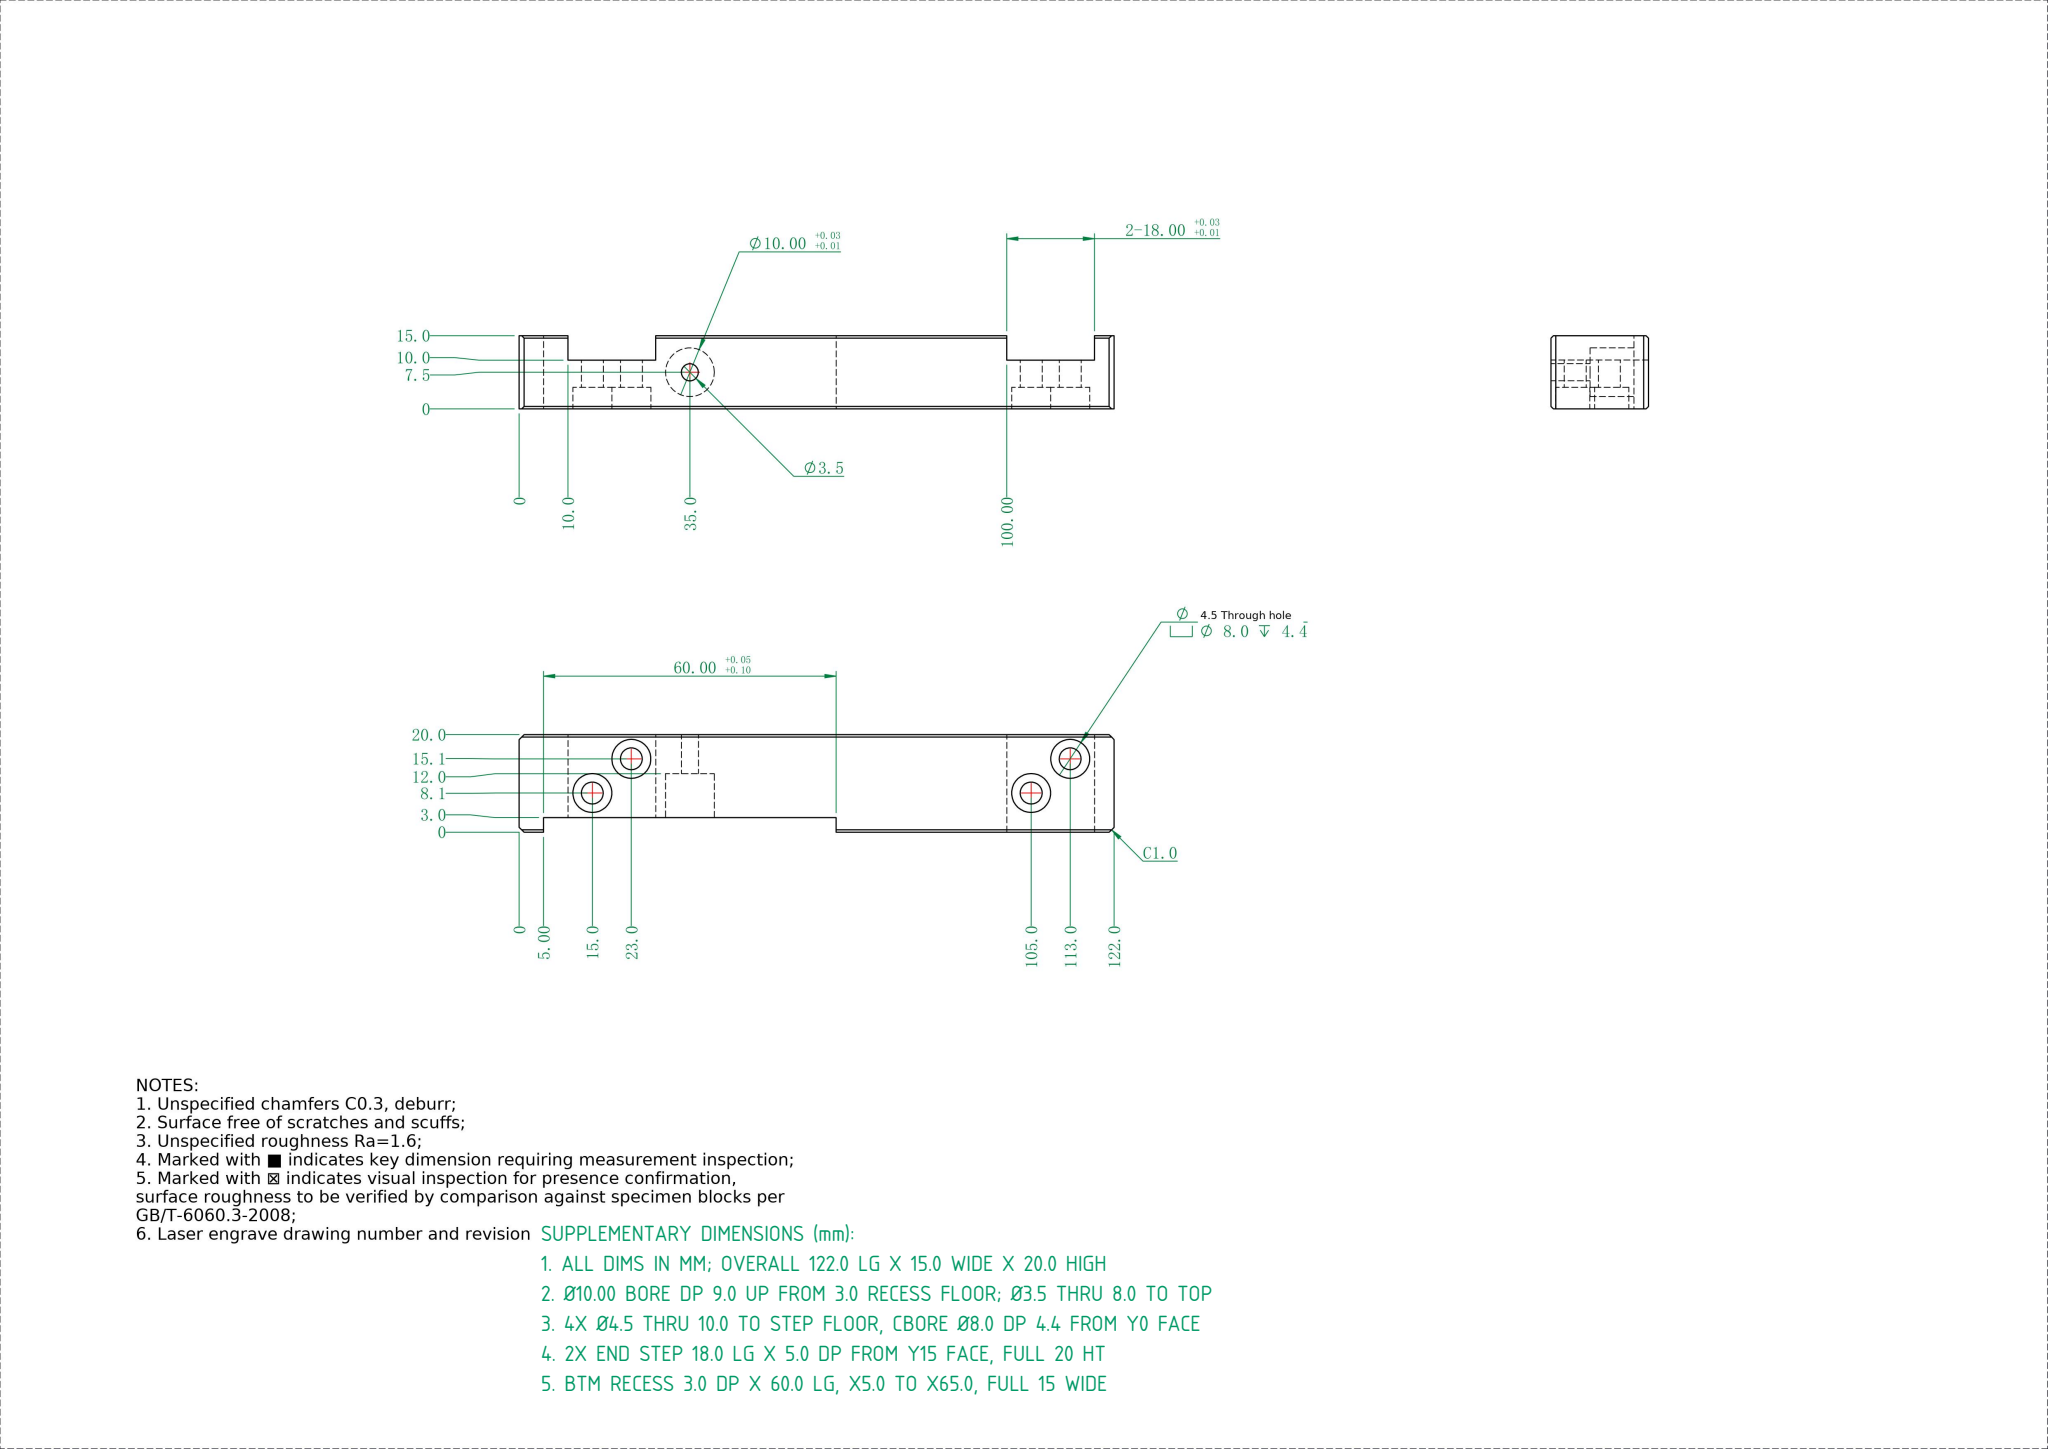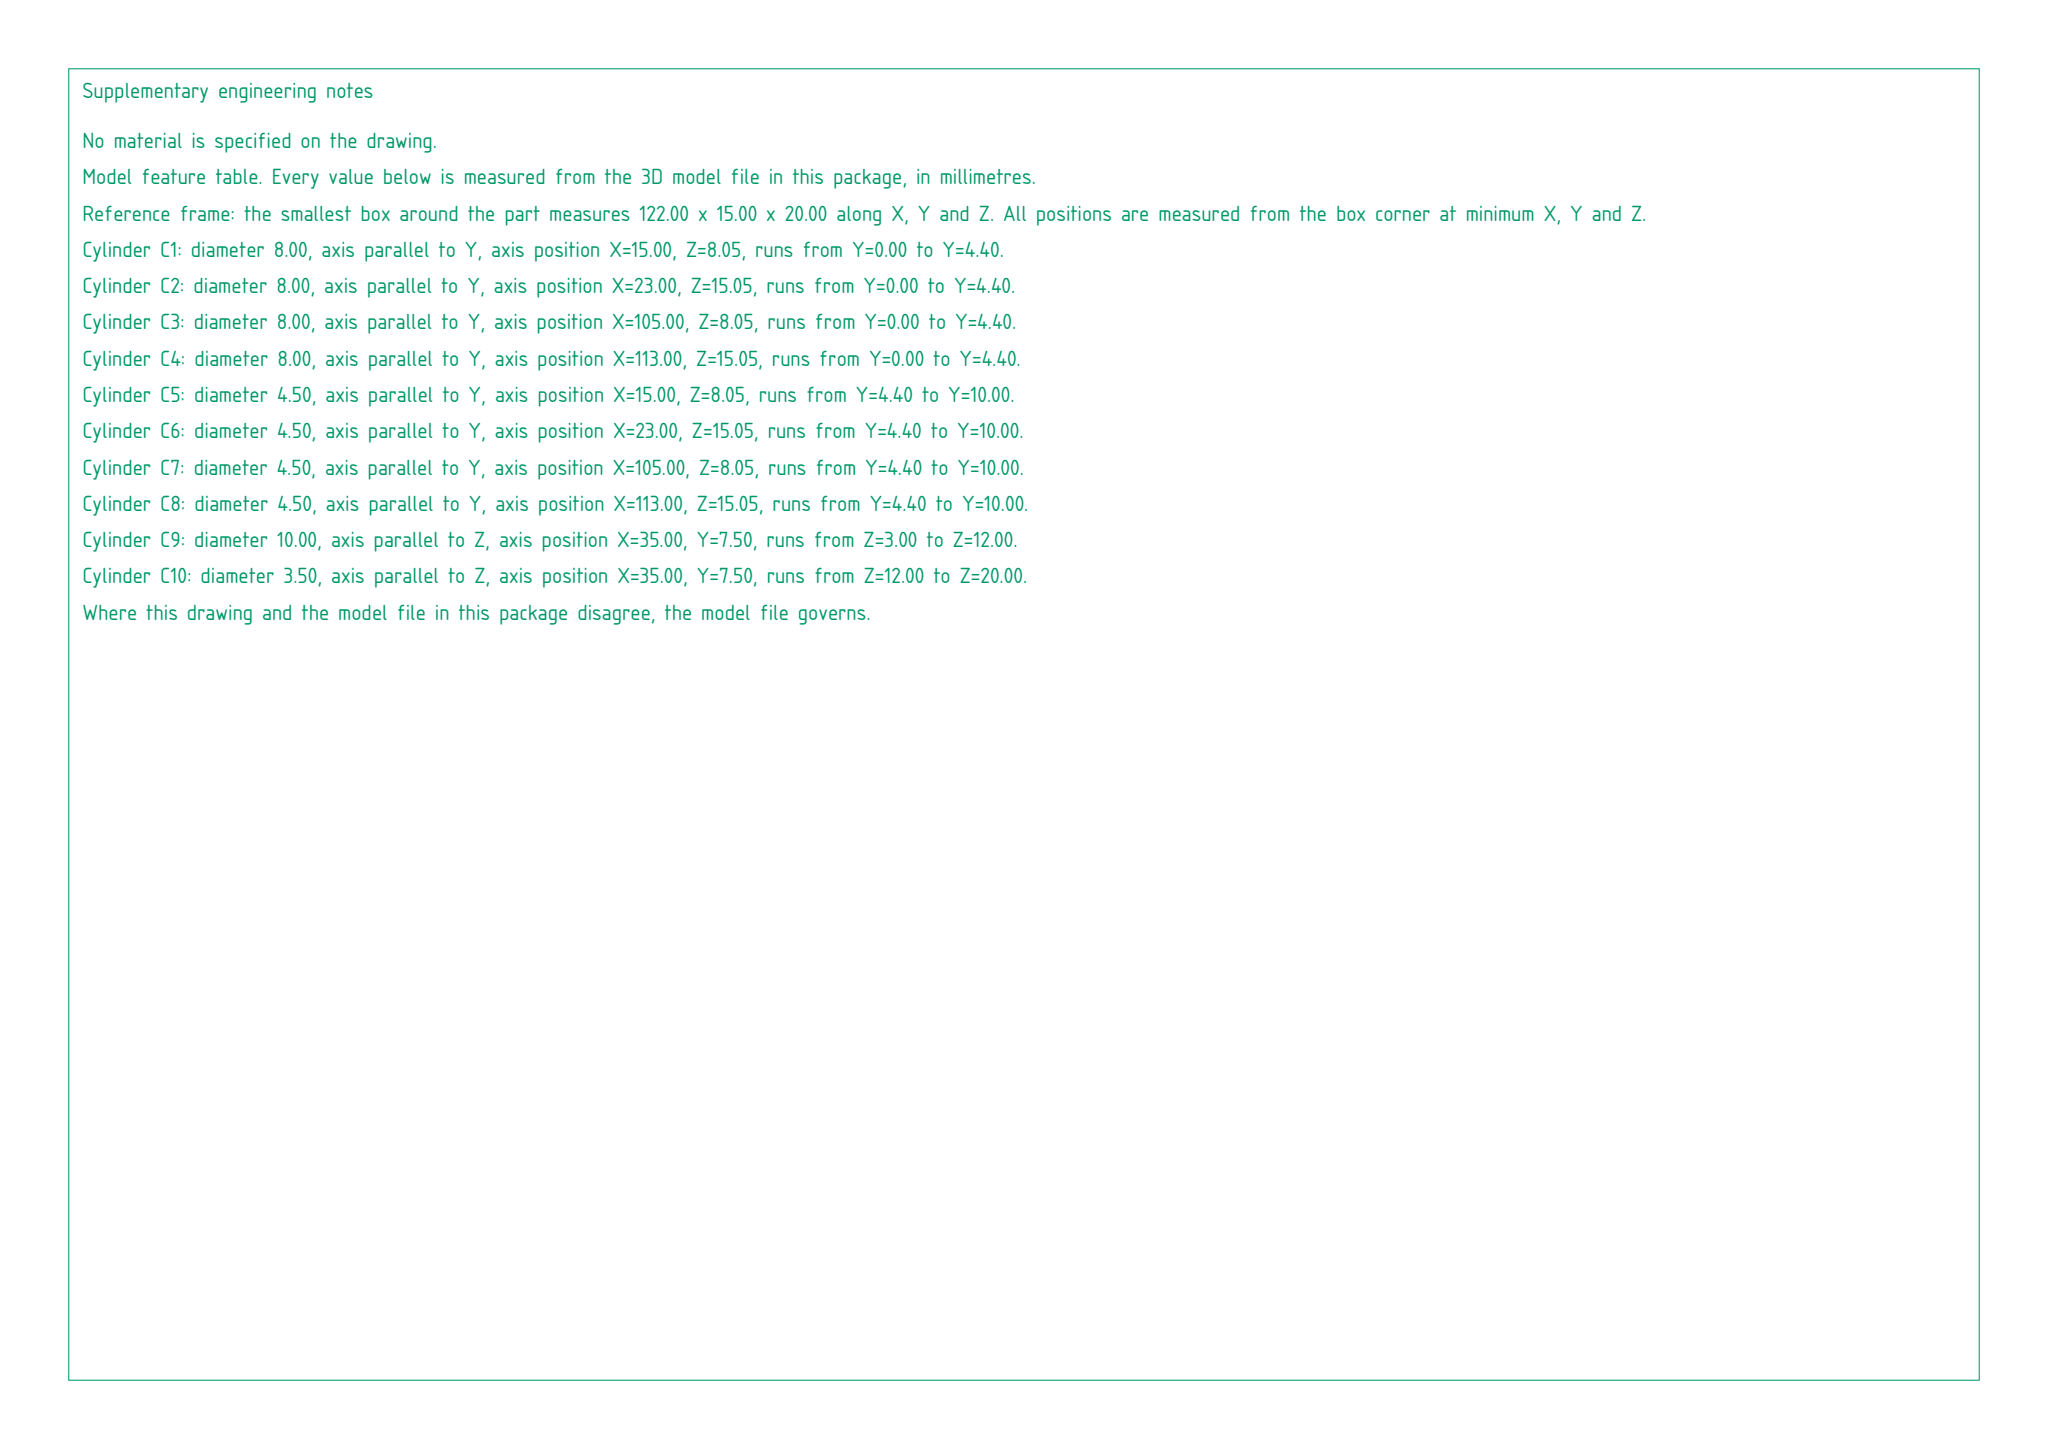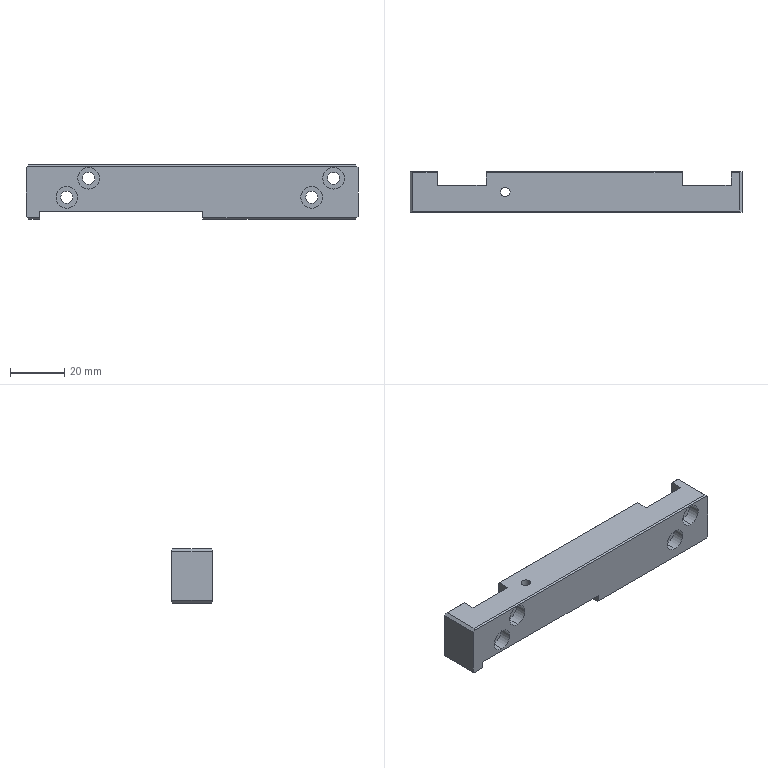Part | SolidWorks | mm | 1 solid | 56 faces | box 122 x 15 x 20 mm | volume 28477 mm3 | plane 36 | cylinder 20 | commonest cylinder face diameters 8 x8 4.5 x8 3.5 x2 10 x2
build123d program:
from build123d import *

# Parameters (mm, degrees)
SKETCH1_W                                       = 122
SKETCH1_H                                       = 15
BOSS_EXTRUDE1_DEPTH                             = 10
SKETCH2_W                                       = 60
SKETCH2_H                                       = 6
CUT_EXTRUDE1_DEPTH                              = 64.608
SKETCH3_R                                       = 5
CUT_EXTRUDE2_DEPTH                              = 64.767
SKETCH4_W                                       = 18
SKETCH4_H                                       = 5
CUT_EXTRUDE3_DEPTH                              = 65.632
BOSS_EXTRUDE2_START                             = -8
SKETCH5_R                                       = 5
SKETCH5_R_2                                     = 1.75
BOSS_EXTRUDE2_DEPTH                             = 8
M4_HEX_SOCKET_HEAD_CAP_SCREW_CBORE1_D           = 4.5
M4_HEX_SOCKET_HEAD_CAP_SCREW_CBORE1_CBORE_D     = 8
M4_HEX_SOCKET_HEAD_CAP_SCREW_CBORE1_CBORE_DEPTH = 4.4
CHAMFER1_SIZE                                   = 1
CHAMFER2_SIZE                                   = 0.5


with BuildPart() as part:
    # Sketch1 → Boss-Extrude1 (new, symmetric)
    with BuildSketch(Plane.XY):
        Rectangle(SKETCH1_W, SKETCH1_H)
    extrude(amount=BOSS_EXTRUDE1_DEPTH, both=True)

    # Sketch2 → Cut-Extrude1 (cut, through all)
    with BuildSketch(Plane(origin=(0, -7.5, 0), x_dir=(-1, 0, 0), z_dir=(0, -1, 0))):
        with Locations((26, 10)):
            Rectangle(SKETCH2_W, SKETCH2_H)
    extrude(amount=-CUT_EXTRUDE1_DEPTH, mode=Mode.SUBTRACT)

    # Sketch3 → Cut-Extrude2 (cut, through all)
    with BuildSketch(Plane(origin=(0, 0, -7), x_dir=(-1, 0, 0), z_dir=(0, 0, -1))):
        with Locations((26, 0)):
            Circle(SKETCH3_R)
    extrude(amount=-CUT_EXTRUDE2_DEPTH, mode=Mode.SUBTRACT)

    # Sketch4 → Cut-Extrude3 (cut, through all)
    with BuildSketch(Plane.XY.offset(10)):
        with Locations((-42, 5)):
            Rectangle(SKETCH4_W, SKETCH4_H)
        with Locations((48, 5)):
            Rectangle(SKETCH4_W, SKETCH4_H)
    extrude(amount=-CUT_EXTRUDE3_DEPTH, mode=Mode.SUBTRACT)

    # Sketch5 → Boss-Extrude2 (add)
    with BuildSketch(Plane.XY.offset(10).offset(BOSS_EXTRUDE2_START)):
        with Locations(Location((-26, 0, 0), (0, 0, 180))):
            Circle(SKETCH5_R)
        with Locations((-26, 0)):
            Circle(SKETCH5_R_2, mode=Mode.SUBTRACT)
    extrude(amount=BOSS_EXTRUDE2_DEPTH)

    # M4 Hex Socket Head Cap Screw CBORE1 (through all)
    with Locations(Plane(origin=(0, -7.5, 0), x_dir=(-1, 0, 0), z_dir=(0, -1, 0))):
        with Locations((38, -5.05), (46, 1.95), (-52, -5.05), (-44, 1.95)):
            CounterBoreHole(M4_HEX_SOCKET_HEAD_CAP_SCREW_CBORE1_D / 2, M4_HEX_SOCKET_HEAD_CAP_SCREW_CBORE1_CBORE_D / 2, M4_HEX_SOCKET_HEAD_CAP_SCREW_CBORE1_CBORE_DEPTH)

    # Chamfer1
    chamfer1_edges = [part.edges().sort_by_distance(p)[0] for p in [
        (61, 0, 10),
        (-61, 0, 10),
        (61, 0, -10),
        (-61, 0, -10),
    ]]
    chamfer(chamfer1_edges, length=CHAMFER1_SIZE)

    # Chamfer2
    chamfer2_edges = [part.edges().sort_by_distance(p)[0] for p in [
        (58.5, 7.5, -10),
        (58.5, 7.5, 10),
        (0, -7.5, 10),
        (-58, -7.5, -10),
        (-58, 7.5, -10),
        (32, -7.5, -10),
        (3, 7.5, 10),
        (-55.5, 7.5, 10),
        (21.5, 7.5, -10),
    ]]
    chamfer(chamfer2_edges, length=CHAMFER2_SIZE)


solid = part.part